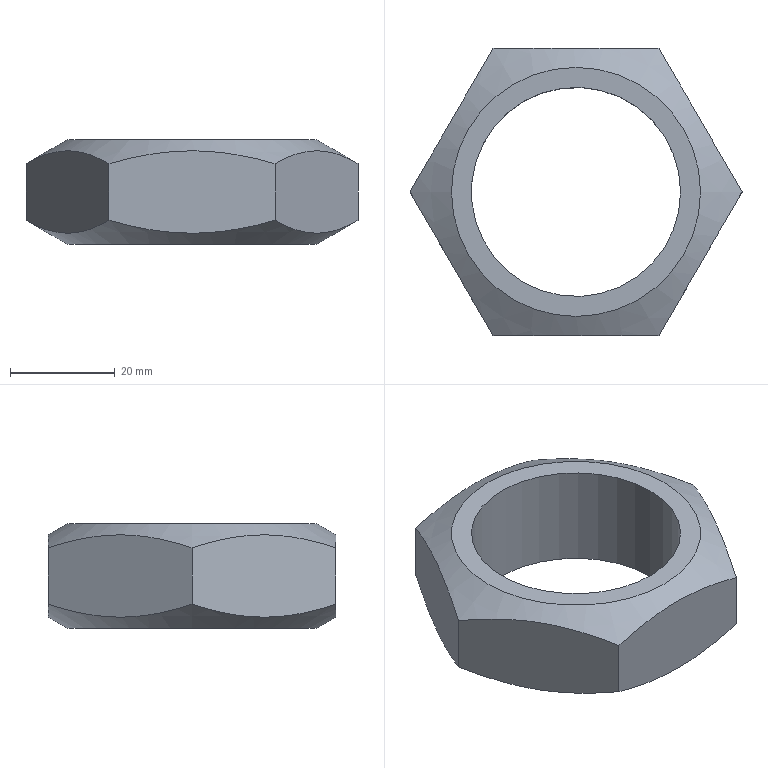Component | NX | NUT | 1 solid | 11 faces | volume 24563 mm3 | plane 8 | cone 2 | cylinder 1 | commonest cylinder face diameters 40 x1